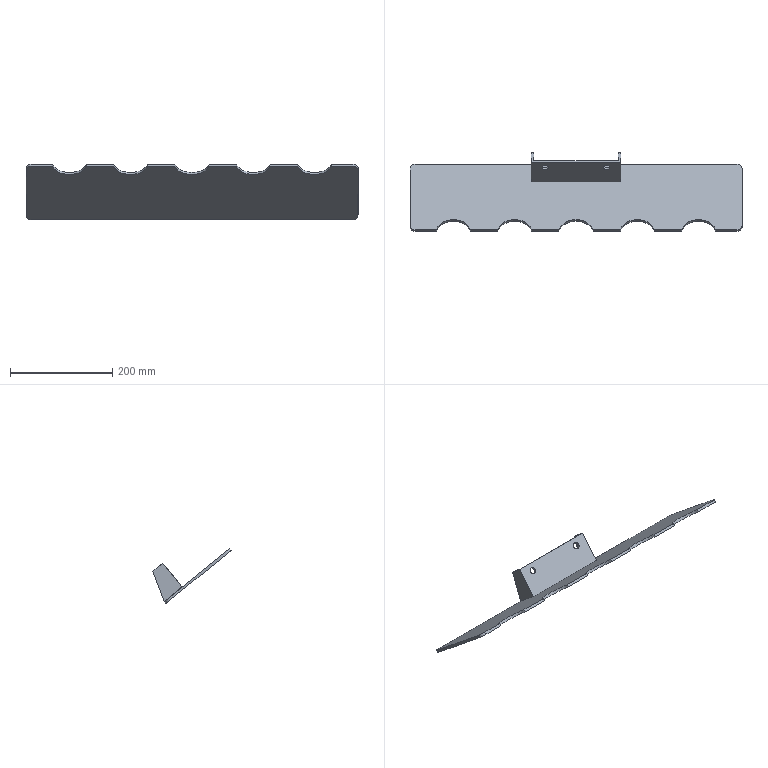Component | SolidWorks | OT-0100-006(MaterialStopBlock)-1 | 1 solid | 34 faces | box 650 x 153.52 x 107.93 mm | volume 574147 mm3 | plane 21 | cylinder 13 | commonest cylinder face diameters 70 x5 13 x4 20 x4 | material AISI 304
STEP:
#1=CARTESIAN_POINT('',(10.492,-3.435,5.002));
#2=VERTEX_POINT('',#1);
#3=CARTESIAN_POINT('',(9.98,-3.435,5.002));
#4=VERTEX_POINT('',#3);
#5=CARTESIAN_POINT('',(10.236,-3.435,5.002));
#6=DIRECTION('',(0.,-0.7761,0.6306));
#7=DIRECTION('',(1.,-0.,-0.));
#8=AXIS2_PLACEMENT_3D('',#5,#6,#7);
#9=CIRCLE('',#8,0.2559);
#10=EDGE_CURVE('',#2,#4,#9,.T.);
#11=ORIENTED_EDGE('',*,*,#10,.T.);
#12=CARTESIAN_POINT('',(9.98,-3.282,4.878));
#13=VERTEX_POINT('',#12);
#14=CARTESIAN_POINT('',(9.98,-7.102,7.981));
#15=DIRECTION('',(-0.,0.7761,-0.6306));
#16=VECTOR('',#15,39.37);
#17=LINE('',#14,#16);
#18=EDGE_CURVE('',#4,#13,#17,.T.);
#19=ORIENTED_EDGE('',*,*,#18,.T.);
#20=CARTESIAN_POINT('',(10.492,-3.282,4.878));
#21=VERTEX_POINT('',#20);
#22=CARTESIAN_POINT('',(10.236,-3.282,4.878));
#23=DIRECTION('',(-0.,0.7761,-0.6306));
#24=DIRECTION('',(-1.,0.,0.));
#25=AXIS2_PLACEMENT_3D('',#22,#23,#24);
#26=CIRCLE('',#25,0.2559);
#27=EDGE_CURVE('',#13,#21,#26,.T.);
#28=ORIENTED_EDGE('',*,*,#27,.T.);
#29=CARTESIAN_POINT('',(10.492,-7.102,7.981));
#30=DIRECTION('',(-0.,0.7761,-0.6306));
#31=VECTOR('',#30,39.37);
#32=LINE('',#29,#31);
#33=EDGE_CURVE('',#2,#21,#32,.T.);
#34=ORIENTED_EDGE('',*,*,#33,.F.);
#35=EDGE_LOOP('',(#11,#19,#28,#34));
#36=FACE_OUTER_BOUND('',#35,.T.);
#37=CARTESIAN_POINT('',(10.236,-7.102,7.981));
#38=DIRECTION('',(-0.,0.7761,-0.6306));
#39=DIRECTION('',(1.,-0.,-0.));
#40=AXIS2_PLACEMENT_3D('',#37,#38,#39);
#41=CYLINDRICAL_SURFACE('',#40,0.2559);
#42=ADVANCED_FACE('',(#36),#41,.F.);
#43=CARTESIAN_POINT('',(5.768,-3.435,5.002));
#44=VERTEX_POINT('',#43);
#45=CARTESIAN_POINT('',(5.256,-3.435,5.002));
#46=VERTEX_POINT('',#45);
#47=CARTESIAN_POINT('',(5.512,-3.435,5.002));
#48=DIRECTION('',(0.,-0.7761,0.6306));
#49=DIRECTION('',(1.,-0.,-0.));
#50=AXIS2_PLACEMENT_3D('',#47,#48,#49);
#51=CIRCLE('',#50,0.2559);
#52=EDGE_CURVE('',#44,#46,#51,.T.);
#53=ORIENTED_EDGE('',*,*,#52,.T.);
#54=CARTESIAN_POINT('',(5.256,-3.282,4.878));
#55=VERTEX_POINT('',#54);
#56=CARTESIAN_POINT('',(5.256,-7.102,7.981));
#57=DIRECTION('',(-0.,0.7761,-0.6306));
#58=VECTOR('',#57,39.37);
#59=LINE('',#56,#58);
#60=EDGE_CURVE('',#46,#55,#59,.T.);
#61=ORIENTED_EDGE('',*,*,#60,.T.);
#62=CARTESIAN_POINT('',(5.768,-3.282,4.878));
#63=VERTEX_POINT('',#62);
#64=CARTESIAN_POINT('',(5.512,-3.282,4.878));
#65=DIRECTION('',(-0.,0.7761,-0.6306));
#66=DIRECTION('',(1.,-0.,-0.));
#67=AXIS2_PLACEMENT_3D('',#64,#65,#66);
#68=CIRCLE('',#67,0.2559);
#69=EDGE_CURVE('',#55,#63,#68,.T.);
#70=ORIENTED_EDGE('',*,*,#69,.T.);
#71=CARTESIAN_POINT('',(5.768,-7.102,7.981));
#72=DIRECTION('',(-0.,0.7761,-0.6306));
#73=VECTOR('',#72,39.37);
#74=LINE('',#71,#73);
#75=EDGE_CURVE('',#44,#63,#74,.T.);
#76=ORIENTED_EDGE('',*,*,#75,.F.);
#77=EDGE_LOOP('',(#53,#61,#70,#76));
#78=FACE_OUTER_BOUND('',#77,.T.);
#79=CARTESIAN_POINT('',(5.512,-7.102,7.981));
#80=DIRECTION('',(-0.,0.7761,-0.6306));
#81=DIRECTION('',(1.,-0.,-0.));
#82=AXIS2_PLACEMENT_3D('',#79,#80,#81);
#83=CYLINDRICAL_SURFACE('',#82,0.2559);
#84=ADVANCED_FACE('',(#78),#83,.F.);
#85=CARTESIAN_POINT('',(4.429,-3.178,2.51));
#86=VERTEX_POINT('',#85);
#87=CARTESIAN_POINT('',(4.429,-4.553,3.627));
#88=VERTEX_POINT('',#87);
#89=CARTESIAN_POINT('',(4.429,-4.553,3.627));
#90=DIRECTION('',(0.,-0.7761,0.6306));
#91=VECTOR('',#90,39.37);
#92=LINE('',#89,#91);
#93=EDGE_CURVE('',#86,#88,#92,.T.);
#94=ORIENTED_EDGE('',*,*,#93,.F.);
#95=CARTESIAN_POINT('',(-4.528,-3.178,2.51));
#96=VERTEX_POINT('',#95);
#97=CARTESIAN_POINT('',(20.669,-3.178,2.51));
#98=DIRECTION('',(1.,-0.,-0.));
#99=VECTOR('',#98,39.37);
#100=LINE('',#97,#99);
#101=EDGE_CURVE('',#96,#86,#100,.T.);
#102=ORIENTED_EDGE('',*,*,#101,.F.);
#103=CARTESIAN_POINT('',(-4.921,-3.483,2.758));
#104=VERTEX_POINT('',#103);
#105=CARTESIAN_POINT('',(-4.528,-3.483,2.758));
#106=DIRECTION('',(0.,0.6306,0.7761));
#107=DIRECTION('',(1.,-0.,-0.));
#108=AXIS2_PLACEMENT_3D('',#105,#106,#107);
#109=CIRCLE('',#108,0.3937);
#110=EDGE_CURVE('',#96,#104,#109,.T.);
#111=ORIENTED_EDGE('',*,*,#110,.T.);
#112=CARTESIAN_POINT('',(-4.921,-7.914,6.358));
#113=VERTEX_POINT('',#112);
#114=CARTESIAN_POINT('',(-4.921,-8.219,6.606));
#115=DIRECTION('',(-0.,0.7761,-0.6306));
#116=VECTOR('',#115,39.37);
#117=LINE('',#114,#116);
#118=EDGE_CURVE('',#113,#104,#117,.T.);
#119=ORIENTED_EDGE('',*,*,#118,.F.);
#120=CARTESIAN_POINT('',(-4.528,-8.219,6.606));
#121=VERTEX_POINT('',#120);
#122=CARTESIAN_POINT('',(-4.528,-7.914,6.358));
#123=DIRECTION('',(0.,0.6306,0.7761));
#124=DIRECTION('',(1.,-0.,-0.));
#125=AXIS2_PLACEMENT_3D('',#122,#123,#124);
#126=CIRCLE('',#125,0.3937);
#127=EDGE_CURVE('',#113,#121,#126,.T.);
#128=ORIENTED_EDGE('',*,*,#127,.T.);
#129=CARTESIAN_POINT('',(-2.895,-8.219,6.606));
#130=VERTEX_POINT('',#129);
#131=CARTESIAN_POINT('',(20.669,-8.219,6.606));
#132=DIRECTION('',(-1.,0.,0.));
#133=VECTOR('',#132,39.37);
#134=LINE('',#131,#133);
#135=EDGE_CURVE('',#130,#121,#134,.T.);
#136=ORIENTED_EDGE('',*,*,#135,.F.);
#137=CARTESIAN_POINT('',(-0.2543,-8.219,6.606));
#138=VERTEX_POINT('',#137);
#139=CARTESIAN_POINT('',(-1.575,-8.525,6.855));
#140=DIRECTION('',(-0.,-0.6306,-0.7761));
#141=DIRECTION('',(-1.,0.,0.));
#142=AXIS2_PLACEMENT_3D('',#139,#140,#141);
#143=CIRCLE('',#142,1.378);
#144=EDGE_CURVE('',#130,#138,#143,.T.);
#145=ORIENTED_EDGE('',*,*,#144,.T.);
#146=CARTESIAN_POINT('',(1.829,-8.219,6.606));
#147=VERTEX_POINT('',#146);
#148=CARTESIAN_POINT('',(20.669,-8.219,6.606));
#149=DIRECTION('',(-1.,0.,0.));
#150=VECTOR('',#149,39.37);
#151=LINE('',#148,#150);
#152=EDGE_CURVE('',#147,#138,#151,.T.);
#153=ORIENTED_EDGE('',*,*,#152,.F.);
#154=CARTESIAN_POINT('',(4.47,-8.219,6.606));
#155=VERTEX_POINT('',#154);
#156=CARTESIAN_POINT('',(3.15,-8.525,6.855));
#157=DIRECTION('',(-0.,-0.6306,-0.7761));
#158=DIRECTION('',(-1.,0.,0.));
#159=AXIS2_PLACEMENT_3D('',#156,#157,#158);
#160=CIRCLE('',#159,1.378);
#161=EDGE_CURVE('',#147,#155,#160,.T.);
#162=ORIENTED_EDGE('',*,*,#161,.T.);
#163=CARTESIAN_POINT('',(6.554,-8.219,6.606));
#164=VERTEX_POINT('',#163);
#165=CARTESIAN_POINT('',(20.669,-8.219,6.606));
#166=DIRECTION('',(-1.,0.,0.));
#167=VECTOR('',#166,39.37);
#168=LINE('',#165,#167);
#169=EDGE_CURVE('',#164,#155,#168,.T.);
#170=ORIENTED_EDGE('',*,*,#169,.F.);
#171=CARTESIAN_POINT('',(9.195,-8.219,6.606));
#172=VERTEX_POINT('',#171);
#173=CARTESIAN_POINT('',(7.874,-8.525,6.855));
#174=DIRECTION('',(-0.,-0.6306,-0.7761));
#175=DIRECTION('',(-1.,0.,0.));
#176=AXIS2_PLACEMENT_3D('',#173,#174,#175);
#177=CIRCLE('',#176,1.378);
#178=EDGE_CURVE('',#164,#172,#177,.T.);
#179=ORIENTED_EDGE('',*,*,#178,.T.);
#180=CARTESIAN_POINT('',(11.278,-8.219,6.606));
#181=VERTEX_POINT('',#180);
#182=CARTESIAN_POINT('',(20.669,-8.219,6.606));
#183=DIRECTION('',(-1.,0.,0.));
#184=VECTOR('',#183,39.37);
#185=LINE('',#182,#184);
#186=EDGE_CURVE('',#181,#172,#185,.T.);
#187=ORIENTED_EDGE('',*,*,#186,.F.);
#188=CARTESIAN_POINT('',(13.919,-8.219,6.606));
#189=VERTEX_POINT('',#188);
#190=CARTESIAN_POINT('',(12.598,-8.525,6.855));
#191=DIRECTION('',(-0.,-0.6306,-0.7761));
#192=DIRECTION('',(1.,-0.,-0.));
#193=AXIS2_PLACEMENT_3D('',#190,#191,#192);
#194=CIRCLE('',#193,1.378);
#195=EDGE_CURVE('',#181,#189,#194,.T.);
#196=ORIENTED_EDGE('',*,*,#195,.T.);
#197=CARTESIAN_POINT('',(16.002,-8.219,6.606));
#198=VERTEX_POINT('',#197);
#199=CARTESIAN_POINT('',(20.669,-8.219,6.606));
#200=DIRECTION('',(-1.,0.,0.));
#201=VECTOR('',#200,39.37);
#202=LINE('',#199,#201);
#203=EDGE_CURVE('',#198,#189,#202,.T.);
#204=ORIENTED_EDGE('',*,*,#203,.F.);
#205=CARTESIAN_POINT('',(18.643,-8.219,6.606));
#206=VERTEX_POINT('',#205);
#207=CARTESIAN_POINT('',(17.323,-8.525,6.855));
#208=DIRECTION('',(-0.,-0.6306,-0.7761));
#209=DIRECTION('',(1.,-0.,-0.));
#210=AXIS2_PLACEMENT_3D('',#207,#208,#209);
#211=CIRCLE('',#210,1.378);
#212=EDGE_CURVE('',#198,#206,#211,.T.);
#213=ORIENTED_EDGE('',*,*,#212,.T.);
#214=CARTESIAN_POINT('',(20.276,-8.219,6.606));
#215=VERTEX_POINT('',#214);
#216=CARTESIAN_POINT('',(20.669,-8.219,6.606));
#217=DIRECTION('',(-1.,0.,0.));
#218=VECTOR('',#217,39.37);
#219=LINE('',#216,#218);
#220=EDGE_CURVE('',#215,#206,#219,.T.);
#221=ORIENTED_EDGE('',*,*,#220,.F.);
#222=CARTESIAN_POINT('',(20.669,-7.914,6.358));
#223=VERTEX_POINT('',#222);
#224=CARTESIAN_POINT('',(20.276,-7.914,6.358));
#225=DIRECTION('',(0.,0.6306,0.7761));
#226=DIRECTION('',(1.,-0.,-0.));
#227=AXIS2_PLACEMENT_3D('',#224,#225,#226);
#228=CIRCLE('',#227,0.3937);
#229=EDGE_CURVE('',#215,#223,#228,.T.);
#230=ORIENTED_EDGE('',*,*,#229,.T.);
#231=CARTESIAN_POINT('',(20.669,-3.483,2.758));
#232=VERTEX_POINT('',#231);
#233=CARTESIAN_POINT('',(20.669,-8.219,6.606));
#234=DIRECTION('',(0.,-0.7761,0.6306));
#235=VECTOR('',#234,39.37);
#236=LINE('',#233,#235);
#237=EDGE_CURVE('',#232,#223,#236,.T.);
#238=ORIENTED_EDGE('',*,*,#237,.F.);
#239=CARTESIAN_POINT('',(20.276,-3.178,2.51));
#240=VERTEX_POINT('',#239);
#241=CARTESIAN_POINT('',(20.276,-3.483,2.758));
#242=DIRECTION('',(0.,0.6306,0.7761));
#243=DIRECTION('',(1.,-0.,-0.));
#244=AXIS2_PLACEMENT_3D('',#241,#242,#243);
#245=CIRCLE('',#244,0.3937);
#246=EDGE_CURVE('',#232,#240,#245,.T.);
#247=ORIENTED_EDGE('',*,*,#246,.T.);
#248=CARTESIAN_POINT('',(11.319,-3.178,2.51));
#249=VERTEX_POINT('',#248);
#250=CARTESIAN_POINT('',(20.669,-3.178,2.51));
#251=DIRECTION('',(1.,-0.,-0.));
#252=VECTOR('',#251,39.37);
#253=LINE('',#250,#252);
#254=EDGE_CURVE('',#249,#240,#253,.T.);
#255=ORIENTED_EDGE('',*,*,#254,.F.);
#256=CARTESIAN_POINT('',(11.319,-4.553,3.627));
#257=VERTEX_POINT('',#256);
#258=CARTESIAN_POINT('',(11.319,-4.553,3.627));
#259=DIRECTION('',(-0.,0.7761,-0.6306));
#260=VECTOR('',#259,39.37);
#261=LINE('',#258,#260);
#262=EDGE_CURVE('',#257,#249,#261,.T.);
#263=ORIENTED_EDGE('',*,*,#262,.F.);
#264=CARTESIAN_POINT('',(4.429,-4.553,3.627));
#265=DIRECTION('',(1.,-0.,-0.));
#266=VECTOR('',#265,39.37);
#267=LINE('',#264,#266);
#268=EDGE_CURVE('',#88,#257,#267,.T.);
#269=ORIENTED_EDGE('',*,*,#268,.F.);
#270=EDGE_LOOP('',(#94,#102,#111,#119,#128,#136,#145,#153,#162,#170,#179,#187,#196,#204,#213,#221,#230,#238,#247,#255,#263,#269));
#271=FACE_OUTER_BOUND('',#270,.T.);
#272=CARTESIAN_POINT('',(20.669,-8.219,6.606));
#273=DIRECTION('',(0.,0.6306,0.7761));
#274=DIRECTION('',(1.,-0.,-0.));
#275=AXIS2_PLACEMENT_3D('',#272,#273,#274);
#276=PLANE('',#275);
#277=ADVANCED_FACE('',(#271),#276,.T.);
#278=CARTESIAN_POINT('',(4.626,-3.178,2.51));
#279=VERTEX_POINT('',#278);
#280=CARTESIAN_POINT('',(4.626,-4.4,3.503));
#281=VERTEX_POINT('',#280);
#282=CARTESIAN_POINT('',(4.626,-4.4,3.503));
#283=DIRECTION('',(0.,-0.7761,0.6306));
#284=VECTOR('',#283,39.37);
#285=LINE('',#282,#284);
#286=EDGE_CURVE('',#279,#281,#285,.T.);
#287=ORIENTED_EDGE('',*,*,#286,.T.);
#288=CARTESIAN_POINT('',(11.122,-4.4,3.503));
#289=VERTEX_POINT('',#288);
#290=CARTESIAN_POINT('',(4.429,-4.4,3.503));
#291=DIRECTION('',(-1.,0.,0.));
#292=VECTOR('',#291,39.37);
#293=LINE('',#290,#292);
#294=EDGE_CURVE('',#289,#281,#293,.T.);
#295=ORIENTED_EDGE('',*,*,#294,.F.);
#296=CARTESIAN_POINT('',(11.122,-3.178,2.51));
#297=VERTEX_POINT('',#296);
#298=CARTESIAN_POINT('',(11.122,-3.178,2.51));
#299=DIRECTION('',(-0.,0.7761,-0.6306));
#300=VECTOR('',#299,39.37);
#301=LINE('',#298,#300);
#302=EDGE_CURVE('',#289,#297,#301,.T.);
#303=ORIENTED_EDGE('',*,*,#302,.T.);
#304=CARTESIAN_POINT('',(20.669,-3.178,2.51));
#305=DIRECTION('',(1.,-0.,-0.));
#306=VECTOR('',#305,39.37);
#307=LINE('',#304,#306);
#308=EDGE_CURVE('',#279,#297,#307,.T.);
#309=ORIENTED_EDGE('',*,*,#308,.F.);
#310=EDGE_LOOP('',(#287,#295,#303,#309));
#311=FACE_OUTER_BOUND('',#310,.T.);
#312=CARTESIAN_POINT('',(20.669,-8.219,6.606));
#313=DIRECTION('',(0.,0.6306,0.7761));
#314=DIRECTION('',(1.,-0.,-0.));
#315=AXIS2_PLACEMENT_3D('',#312,#313,#314);
#316=PLANE('',#315);
#317=ADVANCED_FACE('',(#311),#316,.T.);
#318=ORIENTED_EDGE('',*,*,#203,.T.);
#319=CARTESIAN_POINT('',(13.919,-8.343,6.453));
#320=VERTEX_POINT('',#319);
#321=CARTESIAN_POINT('',(13.919,-8.219,6.606));
#322=DIRECTION('',(-0.,-0.6306,-0.7761));
#323=VECTOR('',#322,39.37);
#324=LINE('',#321,#323);
#325=EDGE_CURVE('',#189,#320,#324,.T.);
#326=ORIENTED_EDGE('',*,*,#325,.T.);
#327=CARTESIAN_POINT('',(16.002,-8.343,6.453));
#328=VERTEX_POINT('',#327);
#329=CARTESIAN_POINT('',(20.669,-8.343,6.453));
#330=DIRECTION('',(-1.,0.,0.));
#331=VECTOR('',#330,39.37);
#332=LINE('',#329,#331);
#333=EDGE_CURVE('',#328,#320,#332,.T.);
#334=ORIENTED_EDGE('',*,*,#333,.F.);
#335=CARTESIAN_POINT('',(16.002,-8.219,6.606));
#336=DIRECTION('',(0.,0.6306,0.7761));
#337=VECTOR('',#336,39.37);
#338=LINE('',#335,#337);
#339=EDGE_CURVE('',#328,#198,#338,.T.);
#340=ORIENTED_EDGE('',*,*,#339,.T.);
#341=EDGE_LOOP('',(#318,#326,#334,#340));
#342=FACE_OUTER_BOUND('',#341,.T.);
#343=CARTESIAN_POINT('',(20.669,-8.343,6.453));
#344=DIRECTION('',(-0.,0.7761,-0.6306));
#345=DIRECTION('',(1.,-0.,-0.));
#346=AXIS2_PLACEMENT_3D('',#343,#344,#345);
#347=PLANE('',#346);
#348=ADVANCED_FACE('',(#342),#347,.F.);
#349=CARTESIAN_POINT('',(20.276,-8.343,6.453));
#350=VERTEX_POINT('',#349);
#351=CARTESIAN_POINT('',(18.643,-8.343,6.453));
#352=VERTEX_POINT('',#351);
#353=CARTESIAN_POINT('',(20.669,-8.343,6.453));
#354=DIRECTION('',(-1.,0.,0.));
#355=VECTOR('',#354,39.37);
#356=LINE('',#353,#355);
#357=EDGE_CURVE('',#350,#352,#356,.T.);
#358=ORIENTED_EDGE('',*,*,#357,.F.);
#359=CARTESIAN_POINT('',(20.276,-8.343,6.453));
#360=DIRECTION('',(0.,0.6306,0.7761));
#361=VECTOR('',#360,39.37);
#362=LINE('',#359,#361);
#363=EDGE_CURVE('',#350,#215,#362,.T.);
#364=ORIENTED_EDGE('',*,*,#363,.T.);
#365=ORIENTED_EDGE('',*,*,#220,.T.);
#366=CARTESIAN_POINT('',(18.643,-8.219,6.606));
#367=DIRECTION('',(-0.,-0.6306,-0.7761));
#368=VECTOR('',#367,39.37);
#369=LINE('',#366,#368);
#370=EDGE_CURVE('',#206,#352,#369,.T.);
#371=ORIENTED_EDGE('',*,*,#370,.T.);
#372=EDGE_LOOP('',(#358,#364,#365,#371));
#373=FACE_OUTER_BOUND('',#372,.T.);
#374=CARTESIAN_POINT('',(20.669,-8.343,6.453));
#375=DIRECTION('',(-0.,0.7761,-0.6306));
#376=DIRECTION('',(1.,-0.,-0.));
#377=AXIS2_PLACEMENT_3D('',#374,#375,#376);
#378=PLANE('',#377);
#379=ADVANCED_FACE('',(#373),#378,.F.);
#380=ORIENTED_EDGE('',*,*,#152,.T.);
#381=CARTESIAN_POINT('',(-0.2543,-8.343,6.453));
#382=VERTEX_POINT('',#381);
#383=CARTESIAN_POINT('',(-0.2543,-8.219,6.606));
#384=DIRECTION('',(-0.,-0.6306,-0.7761));
#385=VECTOR('',#384,39.37);
#386=LINE('',#383,#385);
#387=EDGE_CURVE('',#138,#382,#386,.T.);
#388=ORIENTED_EDGE('',*,*,#387,.T.);
#389=CARTESIAN_POINT('',(1.829,-8.343,6.453));
#390=VERTEX_POINT('',#389);
#391=CARTESIAN_POINT('',(20.669,-8.343,6.453));
#392=DIRECTION('',(-1.,0.,0.));
#393=VECTOR('',#392,39.37);
#394=LINE('',#391,#393);
#395=EDGE_CURVE('',#390,#382,#394,.T.);
#396=ORIENTED_EDGE('',*,*,#395,.F.);
#397=CARTESIAN_POINT('',(1.829,-8.219,6.606));
#398=DIRECTION('',(0.,0.6306,0.7761));
#399=VECTOR('',#398,39.37);
#400=LINE('',#397,#399);
#401=EDGE_CURVE('',#390,#147,#400,.T.);
#402=ORIENTED_EDGE('',*,*,#401,.T.);
#403=EDGE_LOOP('',(#380,#388,#396,#402));
#404=FACE_OUTER_BOUND('',#403,.T.);
#405=CARTESIAN_POINT('',(20.669,-8.343,6.453));
#406=DIRECTION('',(-0.,0.7761,-0.6306));
#407=DIRECTION('',(1.,-0.,-0.));
#408=AXIS2_PLACEMENT_3D('',#405,#406,#407);
#409=PLANE('',#408);
#410=ADVANCED_FACE('',(#404),#409,.F.);
#411=ORIENTED_EDGE('',*,*,#169,.T.);
#412=CARTESIAN_POINT('',(4.47,-8.343,6.453));
#413=VERTEX_POINT('',#412);
#414=CARTESIAN_POINT('',(4.47,-8.219,6.606));
#415=DIRECTION('',(-0.,-0.6306,-0.7761));
#416=VECTOR('',#415,39.37);
#417=LINE('',#414,#416);
#418=EDGE_CURVE('',#155,#413,#417,.T.);
#419=ORIENTED_EDGE('',*,*,#418,.T.);
#420=CARTESIAN_POINT('',(6.554,-8.343,6.453));
#421=VERTEX_POINT('',#420);
#422=CARTESIAN_POINT('',(20.669,-8.343,6.453));
#423=DIRECTION('',(-1.,0.,0.));
#424=VECTOR('',#423,39.37);
#425=LINE('',#422,#424);
#426=EDGE_CURVE('',#421,#413,#425,.T.);
#427=ORIENTED_EDGE('',*,*,#426,.F.);
#428=CARTESIAN_POINT('',(6.554,-8.219,6.606));
#429=DIRECTION('',(0.,0.6306,0.7761));
#430=VECTOR('',#429,39.37);
#431=LINE('',#428,#430);
#432=EDGE_CURVE('',#421,#164,#431,.T.);
#433=ORIENTED_EDGE('',*,*,#432,.T.);
#434=EDGE_LOOP('',(#411,#419,#427,#433));
#435=FACE_OUTER_BOUND('',#434,.T.);
#436=CARTESIAN_POINT('',(20.669,-8.343,6.453));
#437=DIRECTION('',(-0.,0.7761,-0.6306));
#438=DIRECTION('',(1.,-0.,-0.));
#439=AXIS2_PLACEMENT_3D('',#436,#437,#438);
#440=PLANE('',#439);
#441=ADVANCED_FACE('',(#435),#440,.F.);
#442=CARTESIAN_POINT('',(11.278,-8.343,6.453));
#443=VERTEX_POINT('',#442);
#444=CARTESIAN_POINT('',(9.195,-8.343,6.453));
#445=VERTEX_POINT('',#444);
#446=CARTESIAN_POINT('',(20.669,-8.343,6.453));
#447=DIRECTION('',(-1.,0.,0.));
#448=VECTOR('',#447,39.37);
#449=LINE('',#446,#448);
#450=EDGE_CURVE('',#443,#445,#449,.T.);
#451=ORIENTED_EDGE('',*,*,#450,.F.);
#452=CARTESIAN_POINT('',(11.278,-8.219,6.606));
#453=DIRECTION('',(0.,0.6306,0.7761));
#454=VECTOR('',#453,39.37);
#455=LINE('',#452,#454);
#456=EDGE_CURVE('',#443,#181,#455,.T.);
#457=ORIENTED_EDGE('',*,*,#456,.T.);
#458=ORIENTED_EDGE('',*,*,#186,.T.);
#459=CARTESIAN_POINT('',(9.195,-8.219,6.606));
#460=DIRECTION('',(-0.,-0.6306,-0.7761));
#461=VECTOR('',#460,39.37);
#462=LINE('',#459,#461);
#463=EDGE_CURVE('',#172,#445,#462,.T.);
#464=ORIENTED_EDGE('',*,*,#463,.T.);
#465=EDGE_LOOP('',(#451,#457,#458,#464));
#466=FACE_OUTER_BOUND('',#465,.T.);
#467=CARTESIAN_POINT('',(20.669,-8.343,6.453));
#468=DIRECTION('',(-0.,0.7761,-0.6306));
#469=DIRECTION('',(1.,-0.,-0.));
#470=AXIS2_PLACEMENT_3D('',#467,#468,#469);
#471=PLANE('',#470);
#472=ADVANCED_FACE('',(#466),#471,.F.);
#473=ORIENTED_EDGE('',*,*,#237,.T.);
#474=CARTESIAN_POINT('',(20.669,-8.038,6.205));
#475=VERTEX_POINT('',#474);
#476=CARTESIAN_POINT('',(20.669,-8.038,6.205));
#477=DIRECTION('',(-0.,-0.6306,-0.7761));
#478=VECTOR('',#477,39.37);
#479=LINE('',#476,#478);
#480=EDGE_CURVE('',#223,#475,#479,.T.);
#481=ORIENTED_EDGE('',*,*,#480,.T.);
#482=CARTESIAN_POINT('',(20.669,-3.607,2.605));
#483=VERTEX_POINT('',#482);
#484=CARTESIAN_POINT('',(20.669,-8.343,6.453));
#485=DIRECTION('',(0.,-0.7761,0.6306));
#486=VECTOR('',#485,39.37);
#487=LINE('',#484,#486);
#488=EDGE_CURVE('',#483,#475,#487,.T.);
#489=ORIENTED_EDGE('',*,*,#488,.F.);
#490=CARTESIAN_POINT('',(20.669,-3.607,2.605));
#491=DIRECTION('',(0.,0.6306,0.7761));
#492=VECTOR('',#491,39.37);
#493=LINE('',#490,#492);
#494=EDGE_CURVE('',#483,#232,#493,.T.);
#495=ORIENTED_EDGE('',*,*,#494,.T.);
#496=EDGE_LOOP('',(#473,#481,#489,#495));
#497=FACE_OUTER_BOUND('',#496,.T.);
#498=CARTESIAN_POINT('',(20.669,-8.343,6.453));
#499=DIRECTION('',(-1.,0.,0.));
#500=DIRECTION('',(0.,0.6306,0.7761));
#501=AXIS2_PLACEMENT_3D('',#498,#499,#500);
#502=PLANE('',#501);
#503=ADVANCED_FACE('',(#497),#502,.F.);
#504=ORIENTED_EDGE('',*,*,#135,.T.);
#505=CARTESIAN_POINT('',(-4.528,-8.343,6.453));
#506=VERTEX_POINT('',#505);
#507=CARTESIAN_POINT('',(-4.528,-8.343,6.453));
#508=DIRECTION('',(-0.,-0.6306,-0.7761));
#509=VECTOR('',#508,39.37);
#510=LINE('',#507,#509);
#511=EDGE_CURVE('',#121,#506,#510,.T.);
#512=ORIENTED_EDGE('',*,*,#511,.T.);
#513=CARTESIAN_POINT('',(-2.895,-8.343,6.453));
#514=VERTEX_POINT('',#513);
#515=CARTESIAN_POINT('',(20.669,-8.343,6.453));
#516=DIRECTION('',(-1.,0.,0.));
#517=VECTOR('',#516,39.37);
#518=LINE('',#515,#517);
#519=EDGE_CURVE('',#514,#506,#518,.T.);
#520=ORIENTED_EDGE('',*,*,#519,.F.);
#521=CARTESIAN_POINT('',(-2.895,-8.219,6.606));
#522=DIRECTION('',(0.,0.6306,0.7761));
#523=VECTOR('',#522,39.37);
#524=LINE('',#521,#523);
#525=EDGE_CURVE('',#514,#130,#524,.T.);
#526=ORIENTED_EDGE('',*,*,#525,.T.);
#527=EDGE_LOOP('',(#504,#512,#520,#526));
#528=FACE_OUTER_BOUND('',#527,.T.);
#529=CARTESIAN_POINT('',(20.669,-8.343,6.453));
#530=DIRECTION('',(-0.,0.7761,-0.6306));
#531=DIRECTION('',(1.,-0.,-0.));
#532=AXIS2_PLACEMENT_3D('',#529,#530,#531);
#533=PLANE('',#532);
#534=ADVANCED_FACE('',(#528),#533,.F.);
#535=CARTESIAN_POINT('',(-4.921,-8.038,6.205));
#536=VERTEX_POINT('',#535);
#537=CARTESIAN_POINT('',(-4.921,-3.607,2.605));
#538=VERTEX_POINT('',#537);
#539=CARTESIAN_POINT('',(-4.921,-8.343,6.453));
#540=DIRECTION('',(-0.,0.7761,-0.6306));
#541=VECTOR('',#540,39.37);
#542=LINE('',#539,#541);
#543=EDGE_CURVE('',#536,#538,#542,.T.);
#544=ORIENTED_EDGE('',*,*,#543,.F.);
#545=CARTESIAN_POINT('',(-4.921,-8.038,6.205));
#546=DIRECTION('',(0.,0.6306,0.7761));
#547=VECTOR('',#546,39.37);
#548=LINE('',#545,#547);
#549=EDGE_CURVE('',#536,#113,#548,.T.);
#550=ORIENTED_EDGE('',*,*,#549,.T.);
#551=ORIENTED_EDGE('',*,*,#118,.T.);
#552=CARTESIAN_POINT('',(-4.921,-3.607,2.605));
#553=DIRECTION('',(-0.,-0.6306,-0.7761));
#554=VECTOR('',#553,39.37);
#555=LINE('',#552,#554);
#556=EDGE_CURVE('',#104,#538,#555,.T.);
#557=ORIENTED_EDGE('',*,*,#556,.T.);
#558=EDGE_LOOP('',(#544,#550,#551,#557));
#559=FACE_OUTER_BOUND('',#558,.T.);
#560=CARTESIAN_POINT('',(-4.921,-8.343,6.453));
#561=DIRECTION('',(1.,-0.,-0.));
#562=DIRECTION('',(-0.,-0.6306,-0.7761));
#563=AXIS2_PLACEMENT_3D('',#560,#561,#562);
#564=PLANE('',#563);
#565=ADVANCED_FACE('',(#559),#564,.F.);
#566=CARTESIAN_POINT('',(-4.528,-3.302,2.357));
#567=VERTEX_POINT('',#566);
#568=CARTESIAN_POINT('',(20.276,-3.302,2.357));
#569=VERTEX_POINT('',#568);
#570=CARTESIAN_POINT('',(20.669,-3.302,2.357));
#571=DIRECTION('',(1.,-0.,-0.));
#572=VECTOR('',#571,39.37);
#573=LINE('',#570,#572);
#574=EDGE_CURVE('',#567,#569,#573,.T.);
#575=ORIENTED_EDGE('',*,*,#574,.F.);
#576=CARTESIAN_POINT('',(-4.528,-3.302,2.357));
#577=DIRECTION('',(0.,0.6306,0.7761));
#578=VECTOR('',#577,39.37);
#579=LINE('',#576,#578);
#580=EDGE_CURVE('',#567,#96,#579,.T.);
#581=ORIENTED_EDGE('',*,*,#580,.T.);
#582=ORIENTED_EDGE('',*,*,#101,.T.);
#583=CARTESIAN_POINT('',(4.626,-3.178,2.51));
#584=DIRECTION('',(-1.,0.,0.));
#585=VECTOR('',#584,39.37);
#586=LINE('',#583,#585);
#587=EDGE_CURVE('',#279,#86,#586,.T.);
#588=ORIENTED_EDGE('',*,*,#587,.F.);
#589=ORIENTED_EDGE('',*,*,#308,.T.);
#590=CARTESIAN_POINT('',(11.122,-3.178,2.51));
#591=DIRECTION('',(1.,-0.,-0.));
#592=VECTOR('',#591,39.37);
#593=LINE('',#590,#592);
#594=EDGE_CURVE('',#297,#249,#593,.T.);
#595=ORIENTED_EDGE('',*,*,#594,.T.);
#596=ORIENTED_EDGE('',*,*,#254,.T.);
#597=CARTESIAN_POINT('',(20.276,-3.302,2.357));
#598=DIRECTION('',(-0.,-0.6306,-0.7761));
#599=VECTOR('',#598,39.37);
#600=LINE('',#597,#599);
#601=EDGE_CURVE('',#240,#569,#600,.T.);
#602=ORIENTED_EDGE('',*,*,#601,.T.);
#603=EDGE_LOOP('',(#575,#581,#582,#588,#589,#595,#596,#602));
#604=FACE_OUTER_BOUND('',#603,.T.);
#605=CARTESIAN_POINT('',(20.669,-3.302,2.357));
#606=DIRECTION('',(0.,-0.7761,0.6306));
#607=DIRECTION('',(-1.,0.,0.));
#608=AXIS2_PLACEMENT_3D('',#605,#606,#607);
#609=PLANE('',#608);
#610=ADVANCED_FACE('',(#604),#609,.F.);
#611=ORIENTED_EDGE('',*,*,#519,.T.);
#612=CARTESIAN_POINT('',(-4.528,-8.038,6.205));
#613=DIRECTION('',(-0.,-0.6306,-0.7761));
#614=DIRECTION('',(1.,-0.,-0.));
#615=AXIS2_PLACEMENT_3D('',#612,#613,#614);
#616=CIRCLE('',#615,0.3937);
#617=EDGE_CURVE('',#506,#536,#616,.T.);
#618=ORIENTED_EDGE('',*,*,#617,.T.);
#619=ORIENTED_EDGE('',*,*,#543,.T.);
#620=CARTESIAN_POINT('',(-4.528,-3.607,2.605));
#621=DIRECTION('',(-0.,-0.6306,-0.7761));
#622=DIRECTION('',(1.,-0.,-0.));
#623=AXIS2_PLACEMENT_3D('',#620,#621,#622);
#624=CIRCLE('',#623,0.3937);
#625=EDGE_CURVE('',#538,#567,#624,.T.);
#626=ORIENTED_EDGE('',*,*,#625,.T.);
#627=ORIENTED_EDGE('',*,*,#574,.T.);
#628=CARTESIAN_POINT('',(20.276,-3.607,2.605));
#629=DIRECTION('',(-0.,-0.6306,-0.7761));
#630=DIRECTION('',(1.,-0.,-0.));
#631=AXIS2_PLACEMENT_3D('',#628,#629,#630);
#632=CIRCLE('',#631,0.3937);
#633=EDGE_CURVE('',#569,#483,#632,.T.);
#634=ORIENTED_EDGE('',*,*,#633,.T.);
#635=ORIENTED_EDGE('',*,*,#488,.T.);
#636=CARTESIAN_POINT('',(20.276,-8.038,6.205));
#637=DIRECTION('',(-0.,-0.6306,-0.7761));
#638=DIRECTION('',(1.,-0.,-0.));
#639=AXIS2_PLACEMENT_3D('',#636,#637,#638);
#640=CIRCLE('',#639,0.3937);
#641=EDGE_CURVE('',#475,#350,#640,.T.);
#642=ORIENTED_EDGE('',*,*,#641,.T.);
#643=ORIENTED_EDGE('',*,*,#357,.T.);
#644=CARTESIAN_POINT('',(17.323,-8.649,6.702));
#645=DIRECTION('',(-0.,-0.6306,-0.7761));
#646=DIRECTION('',(1.,-0.,-0.));
#647=AXIS2_PLACEMENT_3D('',#644,#645,#646);
#648=CIRCLE('',#647,1.378);
#649=EDGE_CURVE('',#328,#352,#648,.T.);
#650=ORIENTED_EDGE('',*,*,#649,.F.);
#651=ORIENTED_EDGE('',*,*,#333,.T.);
#652=CARTESIAN_POINT('',(12.598,-8.649,6.702));
#653=DIRECTION('',(-0.,-0.6306,-0.7761));
#654=DIRECTION('',(1.,-0.,-0.));
#655=AXIS2_PLACEMENT_3D('',#652,#653,#654);
#656=CIRCLE('',#655,1.378);
#657=EDGE_CURVE('',#443,#320,#656,.T.);
#658=ORIENTED_EDGE('',*,*,#657,.F.);
#659=ORIENTED_EDGE('',*,*,#450,.T.);
#660=CARTESIAN_POINT('',(7.874,-8.649,6.702));
#661=DIRECTION('',(-0.,-0.6306,-0.7761));
#662=DIRECTION('',(-1.,0.,0.));
#663=AXIS2_PLACEMENT_3D('',#660,#661,#662);
#664=CIRCLE('',#663,1.378);
#665=EDGE_CURVE('',#421,#445,#664,.T.);
#666=ORIENTED_EDGE('',*,*,#665,.F.);
#667=ORIENTED_EDGE('',*,*,#426,.T.);
#668=CARTESIAN_POINT('',(3.15,-8.649,6.702));
#669=DIRECTION('',(-0.,-0.6306,-0.7761));
#670=DIRECTION('',(-1.,0.,0.));
#671=AXIS2_PLACEMENT_3D('',#668,#669,#670);
#672=CIRCLE('',#671,1.378);
#673=EDGE_CURVE('',#390,#413,#672,.T.);
#674=ORIENTED_EDGE('',*,*,#673,.F.);
#675=ORIENTED_EDGE('',*,*,#395,.T.);
#676=CARTESIAN_POINT('',(-1.575,-8.649,6.702));
#677=DIRECTION('',(-0.,-0.6306,-0.7761));
#678=DIRECTION('',(-1.,0.,0.));
#679=AXIS2_PLACEMENT_3D('',#676,#677,#678);
#680=CIRCLE('',#679,1.378);
#681=EDGE_CURVE('',#514,#382,#680,.T.);
#682=ORIENTED_EDGE('',*,*,#681,.F.);
#683=EDGE_LOOP('',(#611,#618,#619,#626,#627,#634,#635,#642,#643,#650,#651,#658,#659,#666,#667,#674,#675,#682));
#684=FACE_OUTER_BOUND('',#683,.T.);
#685=CARTESIAN_POINT('',(20.669,-8.343,6.453));
#686=DIRECTION('',(0.,0.6306,0.7761));
#687=DIRECTION('',(1.,-0.,-0.));
#688=AXIS2_PLACEMENT_3D('',#685,#686,#687);
#689=PLANE('',#688);
#690=ADVANCED_FACE('',(#684),#689,.F.);
#691=ORIENTED_EDGE('',*,*,#178,.F.);
#692=ORIENTED_EDGE('',*,*,#432,.F.);
#693=ORIENTED_EDGE('',*,*,#665,.T.);
#694=ORIENTED_EDGE('',*,*,#463,.F.);
#695=EDGE_LOOP('',(#691,#692,#693,#694));
#696=FACE_OUTER_BOUND('',#695,.T.);
#697=CARTESIAN_POINT('',(7.874,-8.525,6.855));
#698=DIRECTION('',(-0.,-0.6306,-0.7761));
#699=DIRECTION('',(-1.,0.,0.));
#700=AXIS2_PLACEMENT_3D('',#697,#698,#699);
#701=CYLINDRICAL_SURFACE('',#700,1.378);
#702=ADVANCED_FACE('',(#696),#701,.F.);
#703=ORIENTED_EDGE('',*,*,#161,.F.);
#704=ORIENTED_EDGE('',*,*,#401,.F.);
#705=ORIENTED_EDGE('',*,*,#673,.T.);
#706=ORIENTED_EDGE('',*,*,#418,.F.);
#707=EDGE_LOOP('',(#703,#704,#705,#706));
#708=FACE_OUTER_BOUND('',#707,.T.);
#709=CARTESIAN_POINT('',(3.15,-8.525,6.855));
#710=DIRECTION('',(-0.,-0.6306,-0.7761));
#711=DIRECTION('',(-1.,0.,0.));
#712=AXIS2_PLACEMENT_3D('',#709,#710,#711);
#713=CYLINDRICAL_SURFACE('',#712,1.378);
#714=ADVANCED_FACE('',(#708),#713,.F.);
#715=ORIENTED_EDGE('',*,*,#144,.F.);
#716=ORIENTED_EDGE('',*,*,#525,.F.);
#717=ORIENTED_EDGE('',*,*,#681,.T.);
#718=ORIENTED_EDGE('',*,*,#387,.F.);
#719=EDGE_LOOP('',(#715,#716,#717,#718));
#720=FACE_OUTER_BOUND('',#719,.T.);
#721=CARTESIAN_POINT('',(-1.575,-8.525,6.855));
#722=DIRECTION('',(-0.,-0.6306,-0.7761));
#723=DIRECTION('',(-1.,0.,0.));
#724=AXIS2_PLACEMENT_3D('',#721,#722,#723);
#725=CYLINDRICAL_SURFACE('',#724,1.378);
#726=ADVANCED_FACE('',(#720),#725,.F.);
#727=ORIENTED_EDGE('',*,*,#212,.F.);
#728=ORIENTED_EDGE('',*,*,#339,.F.);
#729=ORIENTED_EDGE('',*,*,#649,.T.);
#730=ORIENTED_EDGE('',*,*,#370,.F.);
#731=EDGE_LOOP('',(#727,#728,#729,#730));
#732=FACE_OUTER_BOUND('',#731,.T.);
#733=CARTESIAN_POINT('',(17.323,-8.525,6.855));
#734=DIRECTION('',(-0.,-0.6306,-0.7761));
#735=DIRECTION('',(-1.,0.,0.));
#736=AXIS2_PLACEMENT_3D('',#733,#734,#735);
#737=CYLINDRICAL_SURFACE('',#736,1.378);
#738=ADVANCED_FACE('',(#732),#737,.F.);
#739=ORIENTED_EDGE('',*,*,#195,.F.);
#740=ORIENTED_EDGE('',*,*,#456,.F.);
#741=ORIENTED_EDGE('',*,*,#657,.T.);
#742=ORIENTED_EDGE('',*,*,#325,.F.);
#743=EDGE_LOOP('',(#739,#740,#741,#742));
#744=FACE_OUTER_BOUND('',#743,.T.);
#745=CARTESIAN_POINT('',(12.598,-8.525,6.855));
#746=DIRECTION('',(-0.,-0.6306,-0.7761));
#747=DIRECTION('',(-1.,0.,0.));
#748=AXIS2_PLACEMENT_3D('',#745,#746,#747);
#749=CYLINDRICAL_SURFACE('',#748,1.378);
#750=ADVANCED_FACE('',(#744),#749,.F.);
#751=ORIENTED_EDGE('',*,*,#617,.F.);
#752=ORIENTED_EDGE('',*,*,#511,.F.);
#753=ORIENTED_EDGE('',*,*,#127,.F.);
#754=ORIENTED_EDGE('',*,*,#549,.F.);
#755=EDGE_LOOP('',(#751,#752,#753,#754));
#756=FACE_OUTER_BOUND('',#755,.T.);
#757=CARTESIAN_POINT('',(-4.528,-8.038,6.205));
#758=DIRECTION('',(0.,0.6306,0.7761));
#759=DIRECTION('',(1.,-0.,-0.));
#760=AXIS2_PLACEMENT_3D('',#757,#758,#759);
#761=CYLINDRICAL_SURFACE('',#760,0.3937);
#762=ADVANCED_FACE('',(#756),#761,.T.);
#763=ORIENTED_EDGE('',*,*,#625,.F.);
#764=ORIENTED_EDGE('',*,*,#556,.F.);
#765=ORIENTED_EDGE('',*,*,#110,.F.);
#766=ORIENTED_EDGE('',*,*,#580,.F.);
#767=EDGE_LOOP('',(#763,#764,#765,#766));
#768=FACE_OUTER_BOUND('',#767,.T.);
#769=CARTESIAN_POINT('',(-4.528,-3.607,2.605));
#770=DIRECTION('',(0.,0.6306,0.7761));
#771=DIRECTION('',(1.,-0.,-0.));
#772=AXIS2_PLACEMENT_3D('',#769,#770,#771);
#773=CYLINDRICAL_SURFACE('',#772,0.3937);
#774=ADVANCED_FACE('',(#768),#773,.T.);
#775=ORIENTED_EDGE('',*,*,#641,.F.);
#776=ORIENTED_EDGE('',*,*,#480,.F.);
#777=ORIENTED_EDGE('',*,*,#229,.F.);
#778=ORIENTED_EDGE('',*,*,#363,.F.);
#779=EDGE_LOOP('',(#775,#776,#777,#778));
#780=FACE_OUTER_BOUND('',#779,.T.);
#781=CARTESIAN_POINT('',(20.276,-8.038,6.205));
#782=DIRECTION('',(0.,0.6306,0.7761));
#783=DIRECTION('',(1.,-0.,-0.));
#784=AXIS2_PLACEMENT_3D('',#781,#782,#783);
#785=CYLINDRICAL_SURFACE('',#784,0.3937);
#786=ADVANCED_FACE('',(#780),#785,.T.);
#787=ORIENTED_EDGE('',*,*,#633,.F.);
#788=ORIENTED_EDGE('',*,*,#601,.F.);
#789=ORIENTED_EDGE('',*,*,#246,.F.);
#790=ORIENTED_EDGE('',*,*,#494,.F.);
#791=EDGE_LOOP('',(#787,#788,#789,#790));
#792=FACE_OUTER_BOUND('',#791,.T.);
#793=CARTESIAN_POINT('',(20.276,-3.607,2.605));
#794=DIRECTION('',(0.,0.6306,0.7761));
#795=DIRECTION('',(1.,-0.,-0.));
#796=AXIS2_PLACEMENT_3D('',#793,#794,#795);
#797=CYLINDRICAL_SURFACE('',#796,0.3937);
#798=ADVANCED_FACE('',(#792),#797,.T.);
#799=ORIENTED_EDGE('',*,*,#262,.T.);
#800=CARTESIAN_POINT('',(11.319,-2.299,4.839));
#801=VERTEX_POINT('',#800);
#802=CARTESIAN_POINT('',(11.319,-2.299,4.839));
#803=DIRECTION('',(0.,0.3529,0.9357));
#804=VECTOR('',#803,39.37);
#805=LINE('',#802,#804);
#806=EDGE_CURVE('',#249,#801,#805,.T.);
#807=ORIENTED_EDGE('',*,*,#806,.T.);
#808=CARTESIAN_POINT('',(11.319,-3.063,5.46));
#809=VERTEX_POINT('',#808);
#810=CARTESIAN_POINT('',(11.319,-3.063,5.46));
#811=DIRECTION('',(-0.,0.7761,-0.6306));
#812=VECTOR('',#811,39.37);
#813=LINE('',#810,#812);
#814=EDGE_CURVE('',#809,#801,#813,.T.);
#815=ORIENTED_EDGE('',*,*,#814,.F.);
#816=CARTESIAN_POINT('',(11.319,-3.063,5.46));
#817=DIRECTION('',(-0.,-0.6306,-0.7761));
#818=VECTOR('',#817,39.37);
#819=LINE('',#816,#818);
#820=EDGE_CURVE('',#809,#257,#819,.T.);
#821=ORIENTED_EDGE('',*,*,#820,.T.);
#822=EDGE_LOOP('',(#799,#807,#815,#821));
#823=FACE_OUTER_BOUND('',#822,.T.);
#824=CARTESIAN_POINT('',(11.319,-3.063,5.46));
#825=DIRECTION('',(-1.,0.,0.));
#826=DIRECTION('',(0.,0.6306,0.7761));
#827=AXIS2_PLACEMENT_3D('',#824,#825,#826);
#828=PLANE('',#827);
#829=ADVANCED_FACE('',(#823),#828,.F.);
#830=CARTESIAN_POINT('',(10.236,-3.282,4.878));
#831=DIRECTION('',(-0.,0.7761,-0.6306));
#832=DIRECTION('',(-1.,0.,0.));
#833=AXIS2_PLACEMENT_3D('',#830,#831,#832);
#834=CIRCLE('',#833,0.2559);
#835=EDGE_CURVE('',#21,#13,#834,.T.);
#836=ORIENTED_EDGE('',*,*,#835,.F.);
#837=ORIENTED_EDGE('',*,*,#27,.F.);
#838=EDGE_LOOP('',(#836,#837));
#839=FACE_BOUND('',#838,.T.);
#840=CARTESIAN_POINT('',(5.512,-3.282,4.878));
#841=DIRECTION('',(-0.,0.7761,-0.6306));
#842=DIRECTION('',(1.,-0.,-0.));
#843=AXIS2_PLACEMENT_3D('',#840,#841,#842);
#844=CIRCLE('',#843,0.2559);
#845=EDGE_CURVE('',#63,#55,#844,.T.);
#846=ORIENTED_EDGE('',*,*,#845,.F.);
#847=ORIENTED_EDGE('',*,*,#69,.F.);
#848=EDGE_LOOP('',(#846,#847));
#849=FACE_BOUND('',#848,.T.);
#850=ORIENTED_EDGE('',*,*,#294,.T.);
#851=CARTESIAN_POINT('',(4.626,-2.91,5.336));
#852=VERTEX_POINT('',#851);
#853=CARTESIAN_POINT('',(4.626,-2.91,5.336));
#854=DIRECTION('',(0.,0.6306,0.7761));
#855=VECTOR('',#854,39.37);
#856=LINE('',#853,#855);
#857=EDGE_CURVE('',#281,#852,#856,.T.);
#858=ORIENTED_EDGE('',*,*,#857,.T.);
#859=CARTESIAN_POINT('',(11.122,-2.91,5.336));
#860=VERTEX_POINT('',#859);
#861=CARTESIAN_POINT('',(4.429,-2.91,5.336));
#862=DIRECTION('',(-1.,0.,0.));
#863=VECTOR('',#862,39.37);
#864=LINE('',#861,#863);
#865=EDGE_CURVE('',#860,#852,#864,.T.);
#866=ORIENTED_EDGE('',*,*,#865,.F.);
#867=CARTESIAN_POINT('',(11.122,-4.4,3.503));
#868=DIRECTION('',(-0.,-0.6306,-0.7761));
#869=VECTOR('',#868,39.37);
#870=LINE('',#867,#869);
#871=EDGE_CURVE('',#860,#289,#870,.T.);
#872=ORIENTED_EDGE('',*,*,#871,.T.);
#873=EDGE_LOOP('',(#850,#858,#866,#872));
#874=FACE_OUTER_BOUND('',#873,.T.);
#875=CARTESIAN_POINT('',(4.429,-2.91,5.336));
#876=DIRECTION('',(0.,-0.7761,0.6306));
#877=DIRECTION('',(-1.,0.,0.));
#878=AXIS2_PLACEMENT_3D('',#875,#876,#877);
#879=PLANE('',#878);
#880=ADVANCED_FACE('',(#839,#849,#874),#879,.F.);
#881=ORIENTED_EDGE('',*,*,#93,.T.);
#882=CARTESIAN_POINT('',(4.429,-3.063,5.46));
#883=VERTEX_POINT('',#882);
#884=CARTESIAN_POINT('',(4.429,-3.063,5.46));
#885=DIRECTION('',(-0.,-0.6306,-0.7761));
#886=VECTOR('',#885,39.37);
#887=LINE('',#884,#886);
#888=EDGE_CURVE('',#883,#88,#887,.T.);
#889=ORIENTED_EDGE('',*,*,#888,.F.);
#890=CARTESIAN_POINT('',(4.429,-2.299,4.839));
#891=VERTEX_POINT('',#890);
#892=CARTESIAN_POINT('',(4.429,-3.063,5.46));
#893=DIRECTION('',(0.,-0.7761,0.6306));
#894=VECTOR('',#893,39.37);
#895=LINE('',#892,#894);
#896=EDGE_CURVE('',#891,#883,#895,.T.);
#897=ORIENTED_EDGE('',*,*,#896,.F.);
#898=CARTESIAN_POINT('',(4.429,-3.178,2.51));
#899=DIRECTION('',(-0.,-0.3529,-0.9357));
#900=VECTOR('',#899,39.37);
#901=LINE('',#898,#900);
#902=EDGE_CURVE('',#891,#86,#901,.T.);
#903=ORIENTED_EDGE('',*,*,#902,.T.);
#904=EDGE_LOOP('',(#881,#889,#897,#903));
#905=FACE_OUTER_BOUND('',#904,.T.);
#906=CARTESIAN_POINT('',(4.429,-3.063,5.46));
#907=DIRECTION('',(1.,-0.,-0.));
#908=DIRECTION('',(-0.,-0.6306,-0.7761));
#909=AXIS2_PLACEMENT_3D('',#906,#907,#908);
#910=PLANE('',#909);
#911=ADVANCED_FACE('',(#905),#910,.F.);
#912=ORIENTED_EDGE('',*,*,#10,.F.);
#913=CARTESIAN_POINT('',(10.236,-3.435,5.002));
#914=DIRECTION('',(0.,-0.7761,0.6306));
#915=DIRECTION('',(1.,0.,0.));
#916=AXIS2_PLACEMENT_3D('',#913,#914,#915);
#917=CIRCLE('',#916,0.2559);
#918=EDGE_CURVE('',#4,#2,#917,.T.);
#919=ORIENTED_EDGE('',*,*,#918,.F.);
#920=EDGE_LOOP('',(#912,#919));
#921=FACE_BOUND('',#920,.T.);
#922=ORIENTED_EDGE('',*,*,#52,.F.);
#923=CARTESIAN_POINT('',(5.512,-3.435,5.002));
#924=DIRECTION('',(0.,-0.7761,0.6306));
#925=DIRECTION('',(1.,0.,0.));
#926=AXIS2_PLACEMENT_3D('',#923,#924,#925);
#927=CIRCLE('',#926,0.2559);
#928=EDGE_CURVE('',#46,#44,#927,.T.);
#929=ORIENTED_EDGE('',*,*,#928,.F.);
#930=EDGE_LOOP('',(#922,#929));
#931=FACE_BOUND('',#930,.T.);
#932=ORIENTED_EDGE('',*,*,#268,.T.);
#933=ORIENTED_EDGE('',*,*,#820,.F.);
#934=CARTESIAN_POINT('',(4.429,-3.063,5.46));
#935=DIRECTION('',(1.,-0.,-0.));
#936=VECTOR('',#935,39.37);
#937=LINE('',#934,#936);
#938=EDGE_CURVE('',#883,#809,#937,.T.);
#939=ORIENTED_EDGE('',*,*,#938,.F.);
#940=ORIENTED_EDGE('',*,*,#888,.T.);
#941=EDGE_LOOP('',(#932,#933,#939,#940));
#942=FACE_OUTER_BOUND('',#941,.T.);
#943=CARTESIAN_POINT('',(4.429,-3.063,5.46));
#944=DIRECTION('',(-0.,0.7761,-0.6306));
#945=DIRECTION('',(1.,-0.,-0.));
#946=AXIS2_PLACEMENT_3D('',#943,#944,#945);
#947=PLANE('',#946);
#948=ADVANCED_FACE('',(#921,#931,#942),#947,.F.);
#949=ORIENTED_EDGE('',*,*,#814,.T.);
#950=CARTESIAN_POINT('',(11.122,-2.299,4.839));
#951=VERTEX_POINT('',#950);
#952=CARTESIAN_POINT('',(11.122,-2.299,4.839));
#953=DIRECTION('',(1.,-0.,-0.));
#954=VECTOR('',#953,39.37);
#955=LINE('',#952,#954);
#956=EDGE_CURVE('',#951,#801,#955,.T.);
#957=ORIENTED_EDGE('',*,*,#956,.F.);
#958=CARTESIAN_POINT('',(11.122,-2.91,5.336));
#959=DIRECTION('',(0.,-0.7761,0.6306));
#960=VECTOR('',#959,39.37);
#961=LINE('',#958,#960);
#962=EDGE_CURVE('',#951,#860,#961,.T.);
#963=ORIENTED_EDGE('',*,*,#962,.T.);
#964=ORIENTED_EDGE('',*,*,#865,.T.);
#965=CARTESIAN_POINT('',(4.626,-2.299,4.839));
#966=VERTEX_POINT('',#965);
#967=CARTESIAN_POINT('',(4.626,-2.299,4.839));
#968=DIRECTION('',(-0.,0.7761,-0.6306));
#969=VECTOR('',#968,39.37);
#970=LINE('',#967,#969);
#971=EDGE_CURVE('',#852,#966,#970,.T.);
#972=ORIENTED_EDGE('',*,*,#971,.T.);
#973=CARTESIAN_POINT('',(4.626,-2.299,4.839));
#974=DIRECTION('',(-1.,0.,0.));
#975=VECTOR('',#974,39.37);
#976=LINE('',#973,#975);
#977=EDGE_CURVE('',#966,#891,#976,.T.);
#978=ORIENTED_EDGE('',*,*,#977,.T.);
#979=ORIENTED_EDGE('',*,*,#896,.T.);
#980=ORIENTED_EDGE('',*,*,#938,.T.);
#981=EDGE_LOOP('',(#949,#957,#963,#964,#972,#978,#979,#980));
#982=FACE_OUTER_BOUND('',#981,.T.);
#983=CARTESIAN_POINT('',(20.669,-6.729,8.44));
#984=DIRECTION('',(-0.,-0.6306,-0.7761));
#985=DIRECTION('',(-1.,0.,0.));
#986=AXIS2_PLACEMENT_3D('',#983,#984,#985);
#987=PLANE('',#986);
#988=ADVANCED_FACE('',(#982),#987,.F.);
#989=ORIENTED_EDGE('',*,*,#806,.F.);
#990=ORIENTED_EDGE('',*,*,#594,.F.);
#991=CARTESIAN_POINT('',(11.122,-2.299,4.839));
#992=DIRECTION('',(0.,0.3529,0.9357));
#993=VECTOR('',#992,39.37);
#994=LINE('',#991,#993);
#995=EDGE_CURVE('',#297,#951,#994,.T.);
#996=ORIENTED_EDGE('',*,*,#995,.T.);
#997=ORIENTED_EDGE('',*,*,#956,.T.);
#998=EDGE_LOOP('',(#989,#990,#996,#997));
#999=FACE_OUTER_BOUND('',#998,.T.);
#1000=CARTESIAN_POINT('',(11.122,-2.299,4.839));
#1001=DIRECTION('',(0.,0.9357,-0.3529));
#1002=DIRECTION('',(0.,0.3529,0.9357));
#1003=AXIS2_PLACEMENT_3D('',#1000,#1001,#1002);
#1004=PLANE('',#1003);
#1005=ADVANCED_FACE('',(#999),#1004,.T.);
#1006=ORIENTED_EDGE('',*,*,#871,.F.);
#1007=ORIENTED_EDGE('',*,*,#962,.F.);
#1008=ORIENTED_EDGE('',*,*,#995,.F.);
#1009=ORIENTED_EDGE('',*,*,#302,.F.);
#1010=EDGE_LOOP('',(#1006,#1007,#1008,#1009));
#1011=FACE_OUTER_BOUND('',#1010,.T.);
#1012=CARTESIAN_POINT('',(11.122,-8.219,6.606));
#1013=DIRECTION('',(-1.,0.,0.));
#1014=DIRECTION('',(0.,0.6306,0.7761));
#1015=AXIS2_PLACEMENT_3D('',#1012,#1013,#1014);
#1016=PLANE('',#1015);
#1017=ADVANCED_FACE('',(#1011),#1016,.T.);
#1018=ORIENTED_EDGE('',*,*,#902,.F.);
#1019=ORIENTED_EDGE('',*,*,#977,.F.);
#1020=CARTESIAN_POINT('',(4.626,-3.178,2.51));
#1021=DIRECTION('',(-0.,-0.3529,-0.9357));
#1022=VECTOR('',#1021,39.37);
#1023=LINE('',#1020,#1022);
#1024=EDGE_CURVE('',#966,#279,#1023,.T.);
#1025=ORIENTED_EDGE('',*,*,#1024,.T.);
#1026=ORIENTED_EDGE('',*,*,#587,.T.);
#1027=EDGE_LOOP('',(#1018,#1019,#1025,#1026));
#1028=FACE_OUTER_BOUND('',#1027,.T.);
#1029=CARTESIAN_POINT('',(4.626,-3.178,2.51));
#1030=DIRECTION('',(0.,0.9357,-0.3529));
#1031=DIRECTION('',(0.,0.3529,0.9357));
#1032=AXIS2_PLACEMENT_3D('',#1029,#1030,#1031);
#1033=PLANE('',#1032);
#1034=ADVANCED_FACE('',(#1028),#1033,.T.);
#1035=ORIENTED_EDGE('',*,*,#857,.F.);
#1036=ORIENTED_EDGE('',*,*,#286,.F.);
#1037=ORIENTED_EDGE('',*,*,#1024,.F.);
#1038=ORIENTED_EDGE('',*,*,#971,.F.);
#1039=EDGE_LOOP('',(#1035,#1036,#1037,#1038));
#1040=FACE_OUTER_BOUND('',#1039,.T.);
#1041=CARTESIAN_POINT('',(4.626,-8.219,6.606));
#1042=DIRECTION('',(1.,-0.,-0.));
#1043=DIRECTION('',(-0.,-0.6306,-0.7761));
#1044=AXIS2_PLACEMENT_3D('',#1041,#1042,#1043);
#1045=PLANE('',#1044);
#1046=ADVANCED_FACE('',(#1040),#1045,.T.);
#1047=ORIENTED_EDGE('',*,*,#60,.F.);
#1048=ORIENTED_EDGE('',*,*,#928,.T.);
#1049=ORIENTED_EDGE('',*,*,#75,.T.);
#1050=ORIENTED_EDGE('',*,*,#845,.T.);
#1051=EDGE_LOOP('',(#1047,#1048,#1049,#1050));
#1052=FACE_OUTER_BOUND('',#1051,.T.);
#1053=CARTESIAN_POINT('',(5.512,-7.102,7.981));
#1054=DIRECTION('',(-0.,0.7761,-0.6306));
#1055=DIRECTION('',(1.,-0.,-0.));
#1056=AXIS2_PLACEMENT_3D('',#1053,#1054,#1055);
#1057=CYLINDRICAL_SURFACE('',#1056,0.2559);
#1058=ADVANCED_FACE('',(#1052),#1057,.F.);
#1059=ORIENTED_EDGE('',*,*,#18,.F.);
#1060=ORIENTED_EDGE('',*,*,#918,.T.);
#1061=ORIENTED_EDGE('',*,*,#33,.T.);
#1062=ORIENTED_EDGE('',*,*,#835,.T.);
#1063=EDGE_LOOP('',(#1059,#1060,#1061,#1062));
#1064=FACE_OUTER_BOUND('',#1063,.T.);
#1065=CARTESIAN_POINT('',(10.236,-7.102,7.981));
#1066=DIRECTION('',(-0.,0.7761,-0.6306));
#1067=DIRECTION('',(1.,-0.,-0.));
#1068=AXIS2_PLACEMENT_3D('',#1065,#1066,#1067);
#1069=CYLINDRICAL_SURFACE('',#1068,0.2559);
#1070=ADVANCED_FACE('',(#1064),#1069,.F.);
#1071=CLOSED_SHELL('',(#42,#84,#277,#317,#348,#379,#410,#441,#472,#503,#534,#565,#610,#690,#702,#714,#726,#738,#750,#762,#774,#786,#798,#829,#880,#911,#948,#988,#1005,#1017,#1034,#1046,#1058,#1070));
#1072=MANIFOLD_SOLID_BREP('',#1071);
#1073=CARTESIAN_POINT('',(0.,0.,0.));
#1074=DIRECTION('',(0.,0.,1.));
#1075=DIRECTION('',(1.,0.,0.));
#1076=AXIS2_PLACEMENT_3D('',#1073,#1074,#1075);
#1077=(LENGTH_UNIT()NAMED_UNIT(*)SI_UNIT($,.METRE.));
#1078=LENGTH_MEASURE_WITH_UNIT(LENGTH_MEASURE(0.0254),#1077);
#1079=DIMENSIONAL_EXPONENTS(1.,0.,0.,0.,0.,0.,0.);
#1080=(CONVERSION_BASED_UNIT('',#1078)LENGTH_UNIT()NAMED_UNIT(#1079));
#1081=UNCERTAINTY_MEASURE_WITH_UNIT(LENGTH_MEASURE(0.00001),#1080,'','');
#1082=(NAMED_UNIT(*)PLANE_ANGLE_UNIT()SI_UNIT($,.RADIAN.));
#1083=(NAMED_UNIT(*)SI_UNIT($,.STERADIAN.)SOLID_ANGLE_UNIT());
#1084=(GEOMETRIC_REPRESENTATION_CONTEXT(3)GLOBAL_UNCERTAINTY_ASSIGNED_CONTEXT((#1081))GLOBAL_UNIT_ASSIGNED_CONTEXT((#1080,#1082,#1083))REPRESENTATION_CONTEXT('',''));
#1085=ADVANCED_BREP_SHAPE_REPRESENTATION('',(#1072,#1076),#1084);
#1086=COLOUR_RGB('',0.7922,0.8196,0.9333);
#1087=FILL_AREA_STYLE_COLOUR('',#1086);
#1088=FILL_AREA_STYLE('',(#1087));
#1089=SURFACE_STYLE_FILL_AREA(#1088);
#1090=SURFACE_SIDE_STYLE('',(#1089));
#1091=SURFACE_STYLE_USAGE(.BOTH.,#1090);
#1092=PRESENTATION_STYLE_ASSIGNMENT((#1091));
#1093=STYLED_ITEM('',(#1092),#1072);
#1094=(LENGTH_UNIT()NAMED_UNIT(*)SI_UNIT($,.METRE.));
#1095=LENGTH_MEASURE_WITH_UNIT(LENGTH_MEASURE(0.0254),#1094);
#1096=DIMENSIONAL_EXPONENTS(1.,0.,0.,0.,0.,0.,0.);
#1097=(CONVERSION_BASED_UNIT('',#1095)LENGTH_UNIT()NAMED_UNIT(#1096));
#1098=UNCERTAINTY_MEASURE_WITH_UNIT(LENGTH_MEASURE(0.00001),#1097,'','');
#1099=(NAMED_UNIT(*)PLANE_ANGLE_UNIT()SI_UNIT($,.RADIAN.));
#1100=(NAMED_UNIT(*)SI_UNIT($,.STERADIAN.)SOLID_ANGLE_UNIT());
#1101=(GEOMETRIC_REPRESENTATION_CONTEXT(3)GLOBAL_UNCERTAINTY_ASSIGNED_CONTEXT((#1098))GLOBAL_UNIT_ASSIGNED_CONTEXT((#1097,#1099,#1100))REPRESENTATION_CONTEXT('',''));
#1102=MECHANICAL_DESIGN_GEOMETRIC_PRESENTATION_REPRESENTATION('',(#1093),#1101);
#1103=PRESENTATION_LAYER_ASSIGNMENT('','',(#1093));